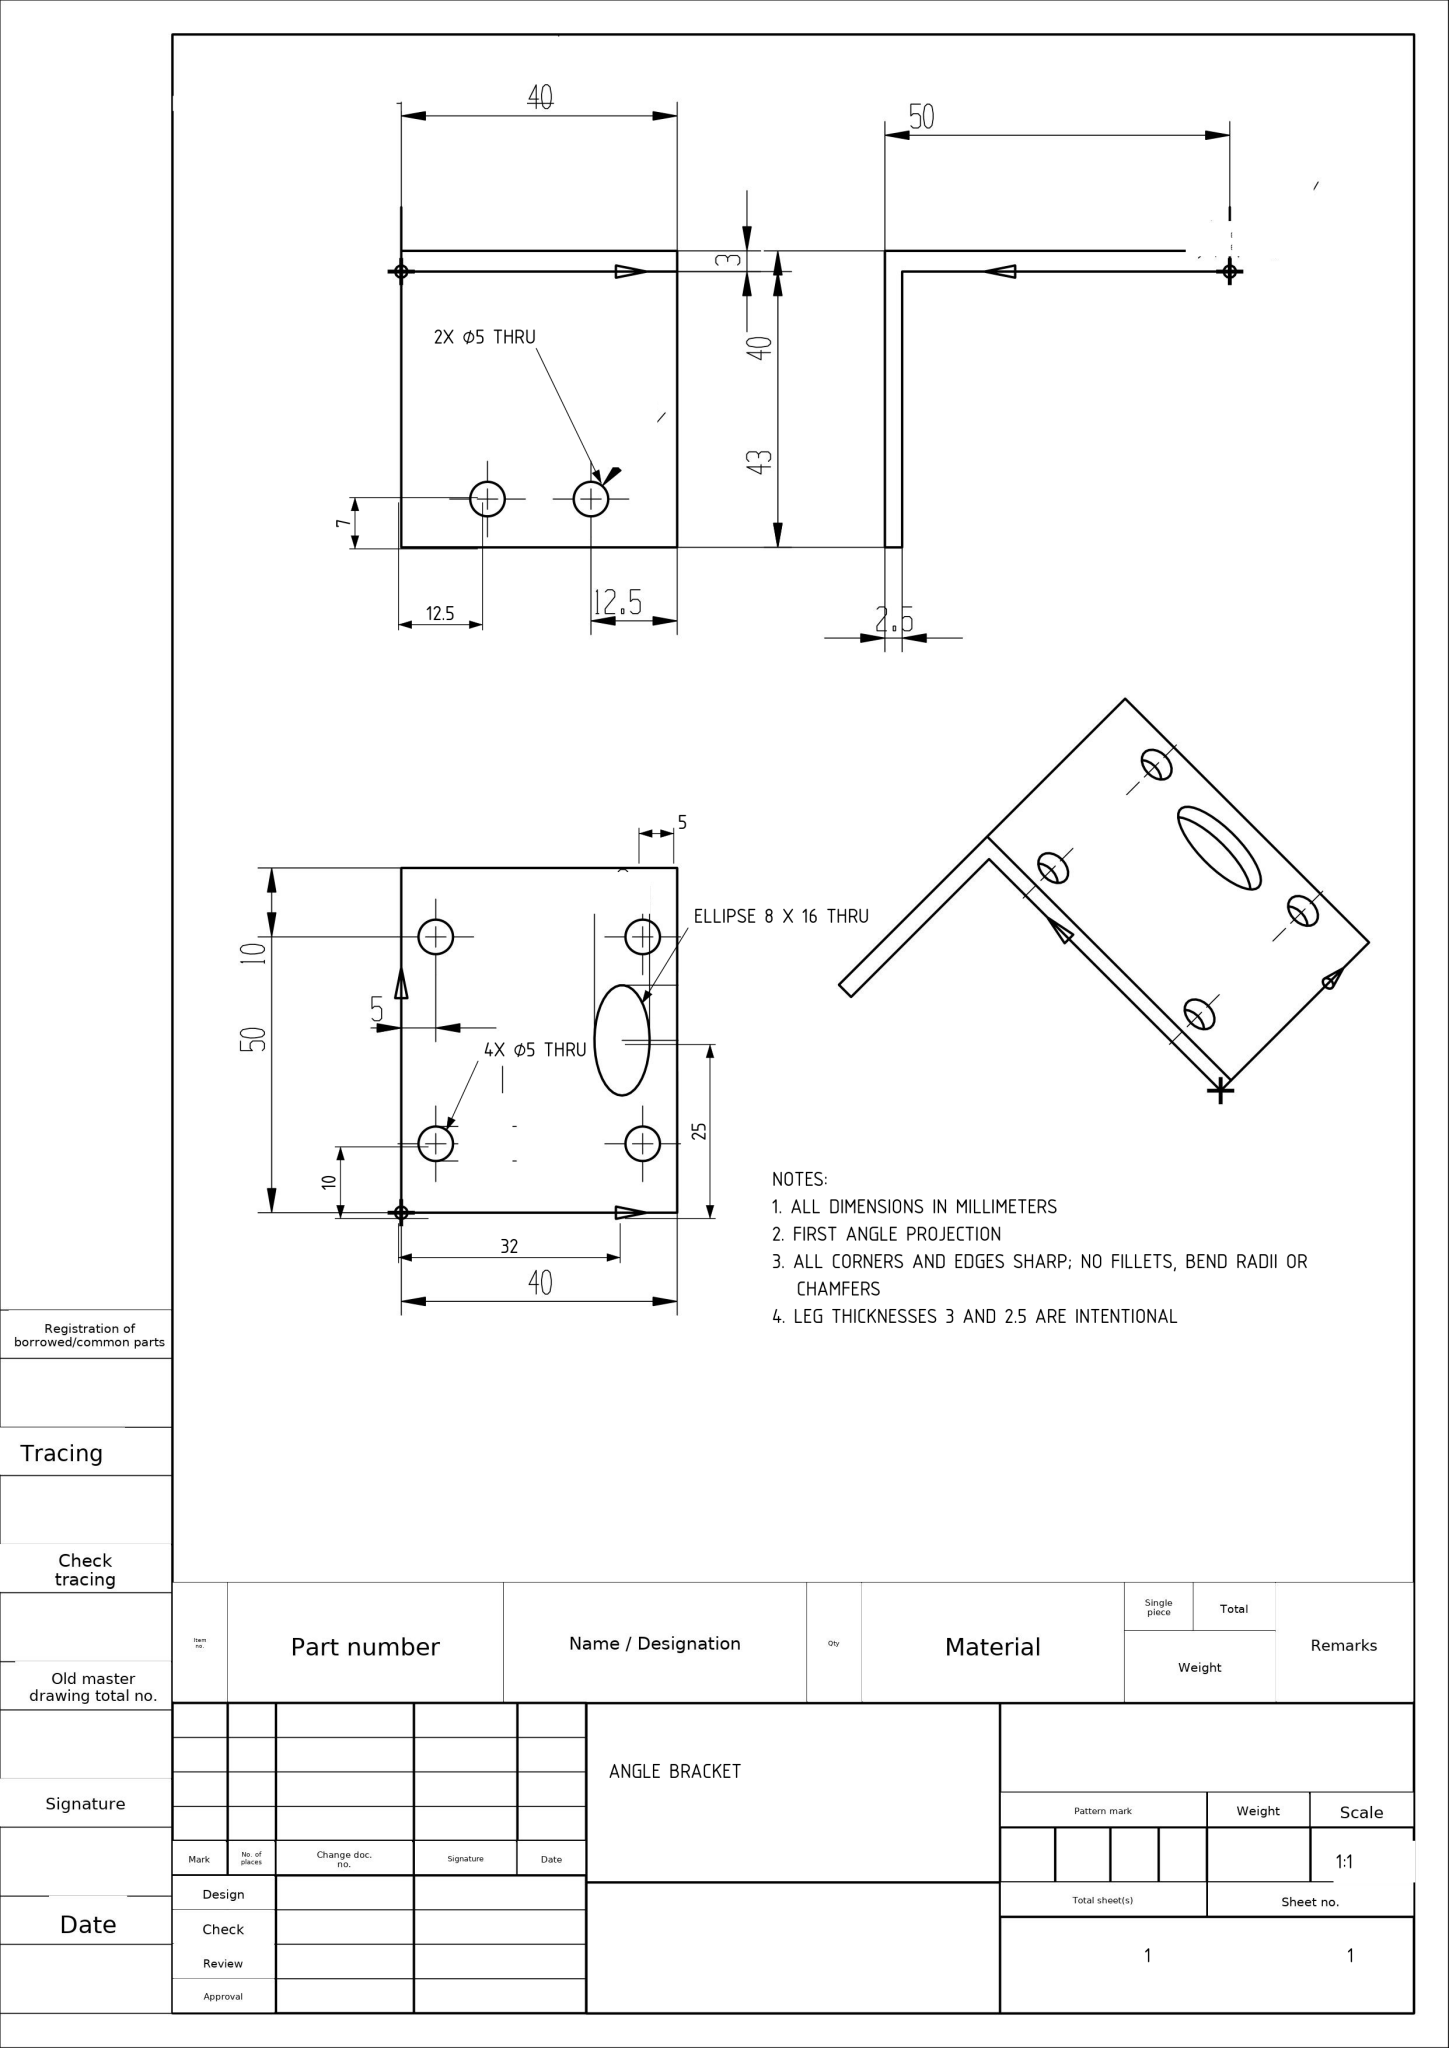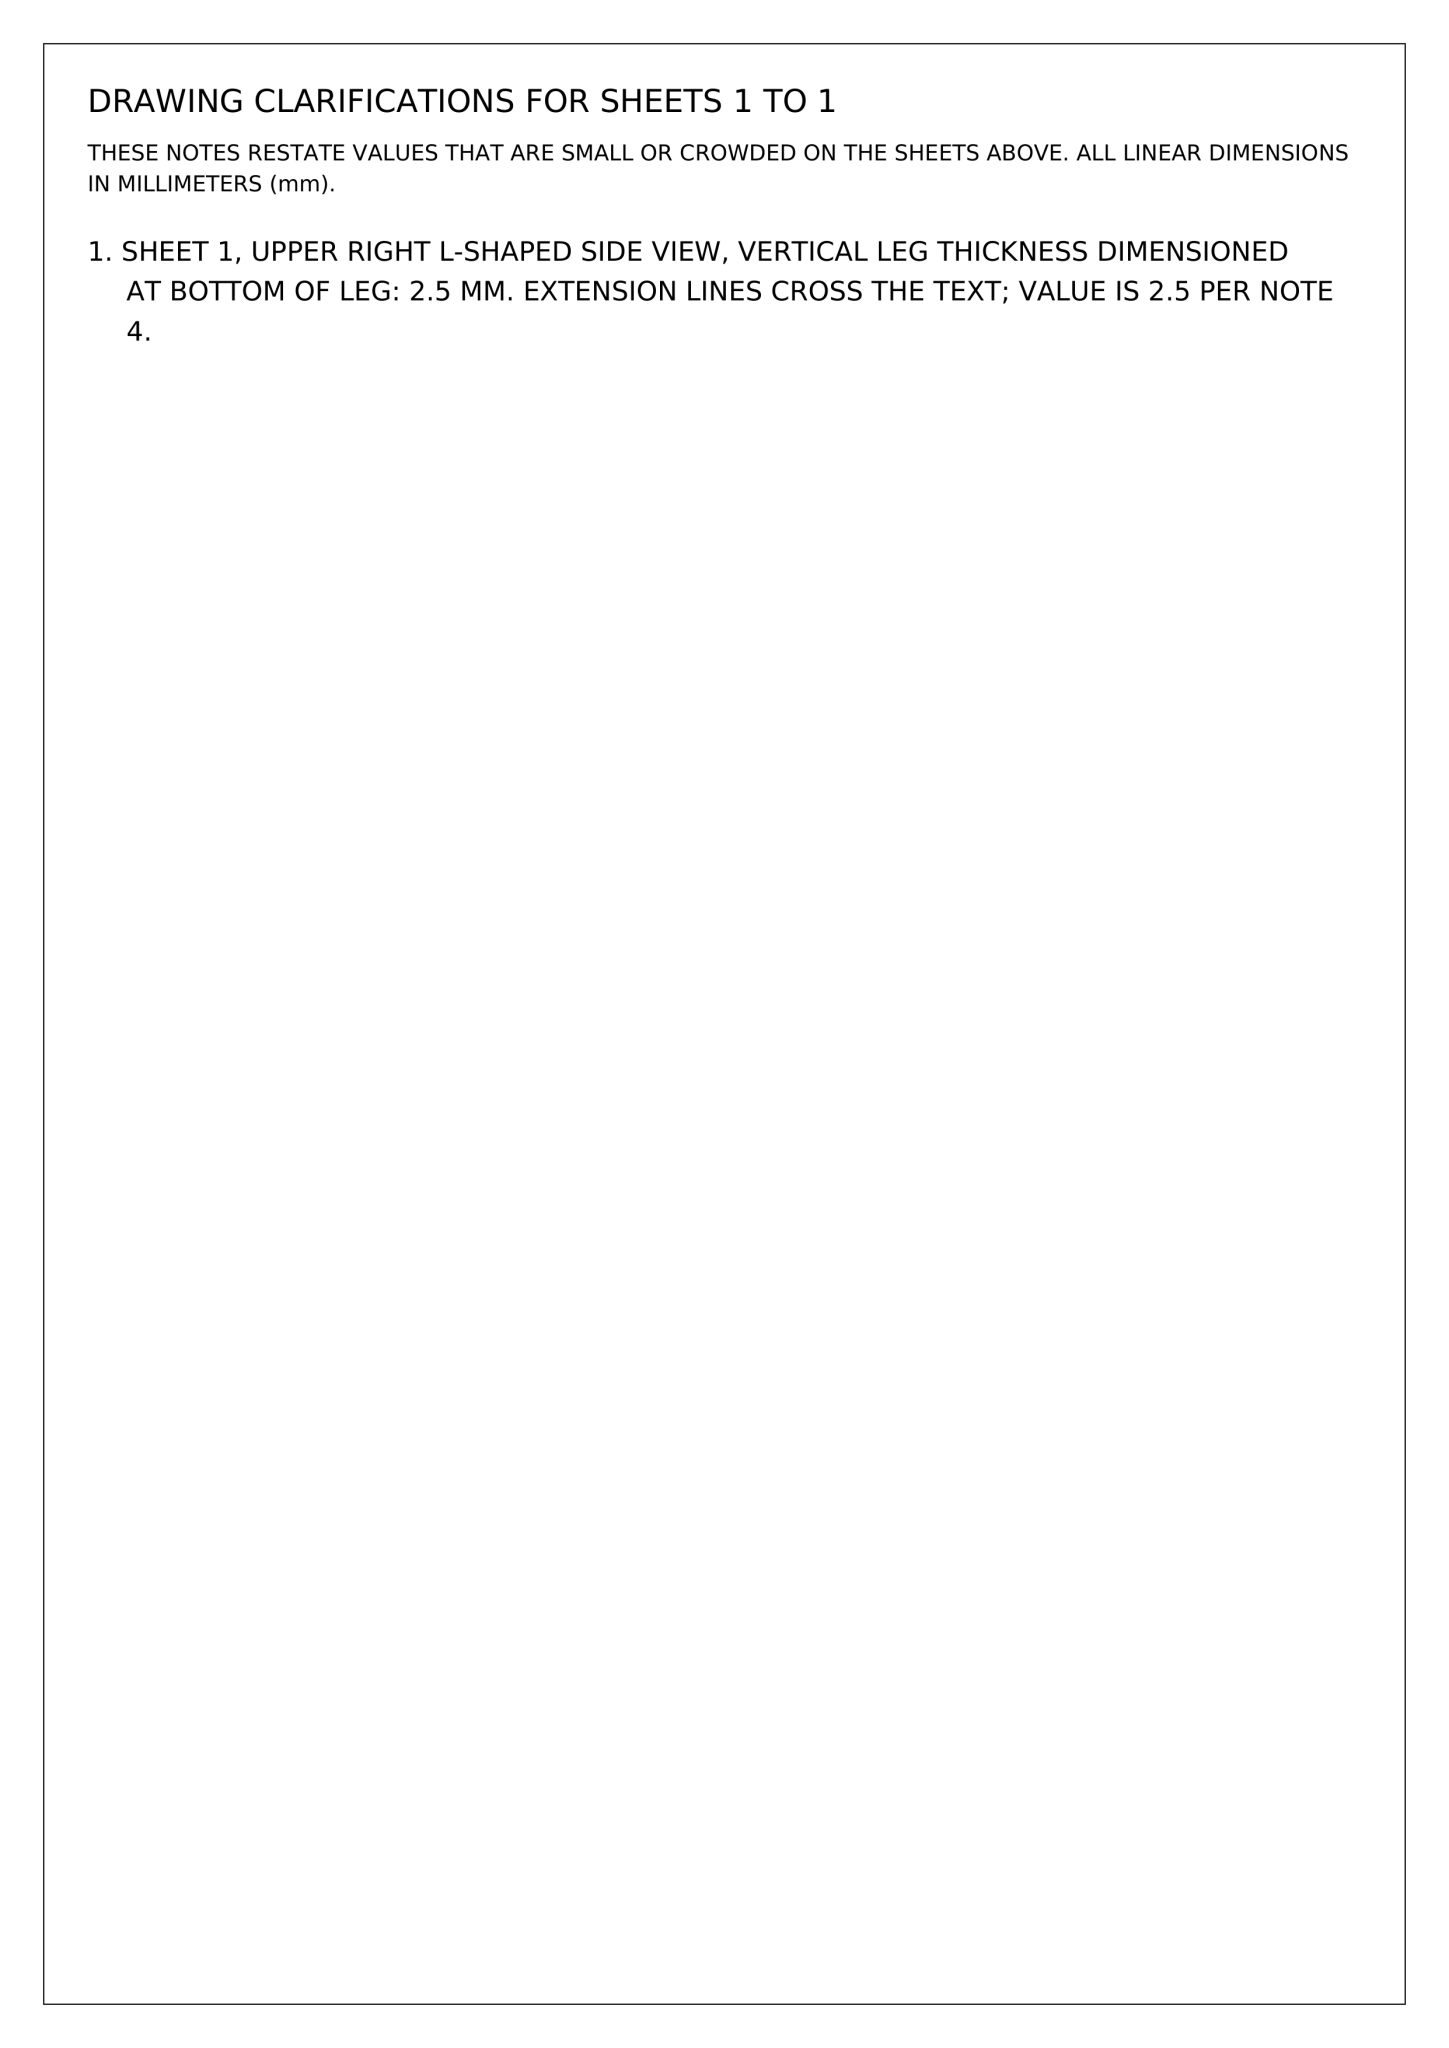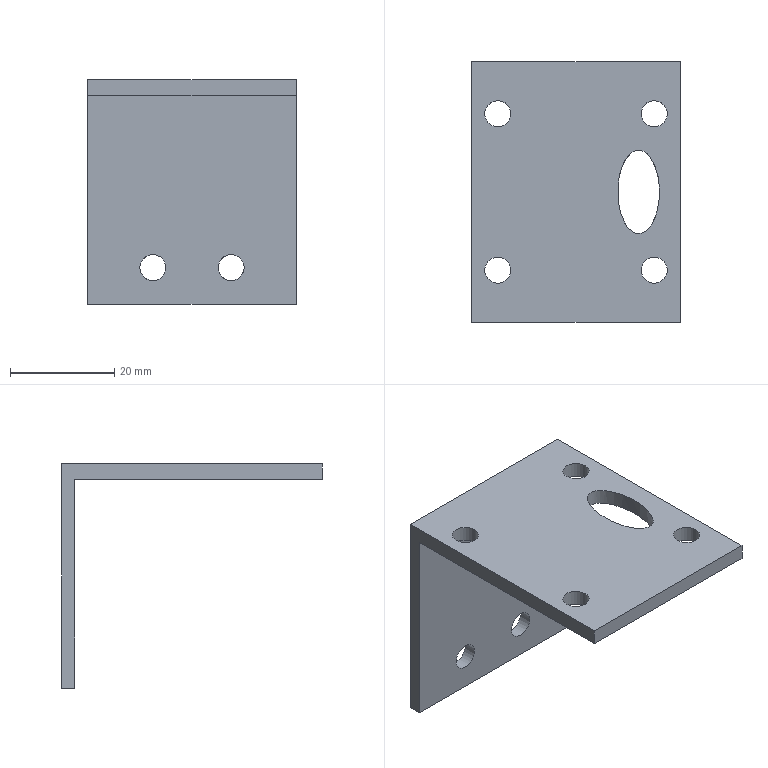Part | NX | mm | 1 solid | 15 faces | box 40 x 50 x 43 mm | volume 9365 mm3 | plane 8 | cylinder 6 | other 1 | commonest cylinder face diameters 5 x6
STEP:
#1=CARTESIAN_POINT('',(0.,0.,0.));
#2=DIRECTION('',(0.,0.,1.));
#3=DIRECTION('',(1.,0.,0.));
#4=AXIS2_PLACEMENT_3D('',#1,#2,#3);
#5=(LENGTH_UNIT()NAMED_UNIT(*)SI_UNIT(.MILLI.,.METRE.));
#6=UNCERTAINTY_MEASURE_WITH_UNIT(LENGTH_MEASURE(0.00002),#5,'','');
#7=(NAMED_UNIT(*)PLANE_ANGLE_UNIT()SI_UNIT($,.RADIAN.));
#8=PLANE_ANGLE_MEASURE_WITH_UNIT(PLANE_ANGLE_MEASURE(0.01745),#7);
#9=DIMENSIONAL_EXPONENTS(0.,0.,0.,0.,0.,0.,0.);
#10=(CONVERSION_BASED_UNIT('',#8)NAMED_UNIT(#9)PLANE_ANGLE_UNIT());
#11=(NAMED_UNIT(*)SI_UNIT($,.STERADIAN.)SOLID_ANGLE_UNIT());
#12=(GEOMETRIC_REPRESENTATION_CONTEXT(3)GLOBAL_UNCERTAINTY_ASSIGNED_CONTEXT((#6))GLOBAL_UNIT_ASSIGNED_CONTEXT((#5,#10,#11))REPRESENTATION_CONTEXT('',''));
#13=SHAPE_REPRESENTATION('',(#4),#12);
#14=CARTESIAN_POINT('',(32.,17.,3.));
#15=VERTEX_POINT('',#14);
#16=CARTESIAN_POINT('',(32.,25.,3.));
#17=DIRECTION('',(0.,0.,1.));
#18=DIRECTION('',(-0.,-1.,0.));
#19=AXIS2_PLACEMENT_3D('',#16,#17,#18);
#20=ELLIPSE('',#19,8.,4.);
#21=EDGE_CURVE('',#15,#15,#20,.T.);
#22=ORIENTED_EDGE('',*,*,#21,.F.);
#23=EDGE_LOOP('',(#22));
#24=FACE_BOUND('',#23,.T.);
#25=CARTESIAN_POINT('',(37.5,40.,3.));
#26=VERTEX_POINT('',#25);
#27=CARTESIAN_POINT('',(35.,40.,3.));
#28=DIRECTION('',(0.,0.,-1.));
#29=DIRECTION('',(1.,0.,0.));
#30=AXIS2_PLACEMENT_3D('',#27,#28,#29);
#31=CIRCLE('',#30,2.5);
#32=EDGE_CURVE('',#26,#26,#31,.T.);
#33=ORIENTED_EDGE('',*,*,#32,.T.);
#34=EDGE_LOOP('',(#33));
#35=FACE_BOUND('',#34,.T.);
#36=CARTESIAN_POINT('',(2.5,10.,3.));
#37=VERTEX_POINT('',#36);
#38=CARTESIAN_POINT('',(5.,10.,3.));
#39=DIRECTION('',(0.,0.,-1.));
#40=DIRECTION('',(-1.,0.,0.));
#41=AXIS2_PLACEMENT_3D('',#38,#39,#40);
#42=CIRCLE('',#41,2.5);
#43=EDGE_CURVE('',#37,#37,#42,.T.);
#44=ORIENTED_EDGE('',*,*,#43,.T.);
#45=EDGE_LOOP('',(#44));
#46=FACE_BOUND('',#45,.T.);
#47=CARTESIAN_POINT('',(40.,0.,3.));
#48=VERTEX_POINT('',#47);
#49=CARTESIAN_POINT('',(0.,0.,3.));
#50=VERTEX_POINT('',#49);
#51=CARTESIAN_POINT('',(20.,0.,3.));
#52=DIRECTION('',(-1.,0.,0.));
#53=VECTOR('',#52,1.);
#54=LINE('',#51,#53);
#55=EDGE_CURVE('',#48,#50,#54,.T.);
#56=ORIENTED_EDGE('',*,*,#55,.F.);
#57=CARTESIAN_POINT('',(40.,50.,3.));
#58=VERTEX_POINT('',#57);
#59=CARTESIAN_POINT('',(40.,25.,3.));
#60=DIRECTION('',(0.,-1.,0.));
#61=VECTOR('',#60,1.);
#62=LINE('',#59,#61);
#63=EDGE_CURVE('',#58,#48,#62,.T.);
#64=ORIENTED_EDGE('',*,*,#63,.F.);
#65=CARTESIAN_POINT('',(0.,50.,3.));
#66=VERTEX_POINT('',#65);
#67=CARTESIAN_POINT('',(20.,50.,3.));
#68=DIRECTION('',(1.,0.,0.));
#69=VECTOR('',#68,1.);
#70=LINE('',#67,#69);
#71=EDGE_CURVE('',#66,#58,#70,.T.);
#72=ORIENTED_EDGE('',*,*,#71,.F.);
#73=CARTESIAN_POINT('',(0.,25.,3.));
#74=DIRECTION('',(0.,1.,0.));
#75=VECTOR('',#74,1.);
#76=LINE('',#73,#75);
#77=EDGE_CURVE('',#50,#66,#76,.T.);
#78=ORIENTED_EDGE('',*,*,#77,.F.);
#79=EDGE_LOOP('',(#56,#64,#72,#78));
#80=FACE_BOUND('',#79,.T.);
#81=CARTESIAN_POINT('',(37.5,10.,3.));
#82=VERTEX_POINT('',#81);
#83=CARTESIAN_POINT('',(35.,10.,3.));
#84=DIRECTION('',(0.,0.,1.));
#85=DIRECTION('',(1.,0.,0.));
#86=AXIS2_PLACEMENT_3D('',#83,#84,#85);
#87=CIRCLE('',#86,2.5);
#88=EDGE_CURVE('',#82,#82,#87,.T.);
#89=ORIENTED_EDGE('',*,*,#88,.F.);
#90=EDGE_LOOP('',(#89));
#91=FACE_BOUND('',#90,.T.);
#92=CARTESIAN_POINT('',(2.5,40.,3.));
#93=VERTEX_POINT('',#92);
#94=CARTESIAN_POINT('',(5.,40.,3.));
#95=DIRECTION('',(0.,0.,1.));
#96=DIRECTION('',(-1.,0.,0.));
#97=AXIS2_PLACEMENT_3D('',#94,#95,#96);
#98=CIRCLE('',#97,2.5);
#99=EDGE_CURVE('',#93,#93,#98,.T.);
#100=ORIENTED_EDGE('',*,*,#99,.F.);
#101=EDGE_LOOP('',(#100));
#102=FACE_BOUND('',#101,.T.);
#103=CARTESIAN_POINT('',(20.,25.,3.));
#104=DIRECTION('',(0.,0.,1.));
#105=DIRECTION('',(1.,0.,0.));
#106=AXIS2_PLACEMENT_3D('',#103,#104,#105);
#107=PLANE('',#106);
#108=ADVANCED_FACE('',(#24,#35,#46,#80,#91,#102),#107,.T.);
#109=CARTESIAN_POINT('',(32.,17.,0.));
#110=VERTEX_POINT('',#109);
#111=CARTESIAN_POINT('',(32.,25.,0.));
#112=DIRECTION('',(0.,0.,-1.));
#113=DIRECTION('',(-0.,-1.,0.));
#114=AXIS2_PLACEMENT_3D('',#111,#112,#113);
#115=ELLIPSE('',#114,8.,4.);
#116=EDGE_CURVE('',#110,#110,#115,.T.);
#117=ORIENTED_EDGE('',*,*,#116,.F.);
#118=EDGE_LOOP('',(#117));
#119=FACE_BOUND('',#118,.T.);
#120=CARTESIAN_POINT('',(40.,47.5,0.));
#121=VERTEX_POINT('',#120);
#122=CARTESIAN_POINT('',(0.,47.5,0.));
#123=VERTEX_POINT('',#122);
#124=CARTESIAN_POINT('',(40.,47.5,0.));
#125=DIRECTION('',(-1.,0.,0.));
#126=VECTOR('',#125,1.);
#127=LINE('',#124,#126);
#128=EDGE_CURVE('',#121,#123,#127,.T.);
#129=ORIENTED_EDGE('',*,*,#128,.F.);
#130=CARTESIAN_POINT('',(40.,0.,0.));
#131=VERTEX_POINT('',#130);
#132=CARTESIAN_POINT('',(40.,25.,0.));
#133=DIRECTION('',(0.,1.,0.));
#134=VECTOR('',#133,1.);
#135=LINE('',#132,#134);
#136=EDGE_CURVE('',#131,#121,#135,.T.);
#137=ORIENTED_EDGE('',*,*,#136,.F.);
#138=CARTESIAN_POINT('',(0.,0.,0.));
#139=VERTEX_POINT('',#138);
#140=CARTESIAN_POINT('',(20.,0.,0.));
#141=DIRECTION('',(1.,0.,0.));
#142=VECTOR('',#141,1.);
#143=LINE('',#140,#142);
#144=EDGE_CURVE('',#139,#131,#143,.T.);
#145=ORIENTED_EDGE('',*,*,#144,.F.);
#146=CARTESIAN_POINT('',(0.,25.,0.));
#147=DIRECTION('',(0.,-1.,0.));
#148=VECTOR('',#147,1.);
#149=LINE('',#146,#148);
#150=EDGE_CURVE('',#123,#139,#149,.T.);
#151=ORIENTED_EDGE('',*,*,#150,.F.);
#152=EDGE_LOOP('',(#129,#137,#145,#151));
#153=FACE_BOUND('',#152,.T.);
#154=CARTESIAN_POINT('',(32.5,40.,0.));
#155=VERTEX_POINT('',#154);
#156=CARTESIAN_POINT('',(35.,40.,0.));
#157=DIRECTION('',(0.,0.,1.));
#158=DIRECTION('',(-1.,0.,0.));
#159=AXIS2_PLACEMENT_3D('',#156,#157,#158);
#160=CIRCLE('',#159,2.5);
#161=EDGE_CURVE('',#155,#155,#160,.T.);
#162=ORIENTED_EDGE('',*,*,#161,.T.);
#163=EDGE_LOOP('',(#162));
#164=FACE_BOUND('',#163,.T.);
#165=CARTESIAN_POINT('',(2.5,10.,0.));
#166=VERTEX_POINT('',#165);
#167=CARTESIAN_POINT('',(5.,10.,0.));
#168=DIRECTION('',(0.,0.,1.));
#169=DIRECTION('',(-1.,0.,0.));
#170=AXIS2_PLACEMENT_3D('',#167,#168,#169);
#171=CIRCLE('',#170,2.5);
#172=EDGE_CURVE('',#166,#166,#171,.T.);
#173=ORIENTED_EDGE('',*,*,#172,.T.);
#174=EDGE_LOOP('',(#173));
#175=FACE_BOUND('',#174,.T.);
#176=CARTESIAN_POINT('',(32.5,10.,0.));
#177=VERTEX_POINT('',#176);
#178=CARTESIAN_POINT('',(35.,10.,0.));
#179=DIRECTION('',(0.,0.,-1.));
#180=DIRECTION('',(-1.,0.,0.));
#181=AXIS2_PLACEMENT_3D('',#178,#179,#180);
#182=CIRCLE('',#181,2.5);
#183=EDGE_CURVE('',#177,#177,#182,.T.);
#184=ORIENTED_EDGE('',*,*,#183,.F.);
#185=EDGE_LOOP('',(#184));
#186=FACE_BOUND('',#185,.T.);
#187=CARTESIAN_POINT('',(2.5,40.,0.));
#188=VERTEX_POINT('',#187);
#189=CARTESIAN_POINT('',(5.,40.,0.));
#190=DIRECTION('',(0.,0.,-1.));
#191=DIRECTION('',(-1.,0.,0.));
#192=AXIS2_PLACEMENT_3D('',#189,#190,#191);
#193=CIRCLE('',#192,2.5);
#194=EDGE_CURVE('',#188,#188,#193,.T.);
#195=ORIENTED_EDGE('',*,*,#194,.F.);
#196=EDGE_LOOP('',(#195));
#197=FACE_BOUND('',#196,.T.);
#198=CARTESIAN_POINT('',(20.,25.,0.));
#199=DIRECTION('',(0.,0.,-1.));
#200=DIRECTION('',(-1.,0.,0.));
#201=AXIS2_PLACEMENT_3D('',#198,#199,#200);
#202=PLANE('',#201);
#203=ADVANCED_FACE('',(#119,#153,#164,#175,#186,#197),#202,.T.);
#204=CARTESIAN_POINT('',(40.,0.,0.));
#205=DIRECTION('',(0.,0.,1.));
#206=VECTOR('',#205,1.);
#207=LINE('',#204,#206);
#208=EDGE_CURVE('',#131,#48,#207,.T.);
#209=ORIENTED_EDGE('',*,*,#208,.T.);
#210=ORIENTED_EDGE('',*,*,#55,.T.);
#211=CARTESIAN_POINT('',(0.,0.,0.));
#212=DIRECTION('',(0.,0.,1.));
#213=VECTOR('',#212,1.);
#214=LINE('',#211,#213);
#215=EDGE_CURVE('',#139,#50,#214,.T.);
#216=ORIENTED_EDGE('',*,*,#215,.F.);
#217=ORIENTED_EDGE('',*,*,#144,.T.);
#218=EDGE_LOOP('',(#209,#210,#216,#217));
#219=FACE_OUTER_BOUND('',#218,.T.);
#220=CARTESIAN_POINT('',(20.,0.,0.));
#221=DIRECTION('',(0.,-1.,0.));
#222=DIRECTION('',(0.,0.,-1.));
#223=AXIS2_PLACEMENT_3D('',#220,#221,#222);
#224=PLANE('',#223);
#225=ADVANCED_FACE('',(#219),#224,.T.);
#226=ORIENTED_EDGE('',*,*,#215,.T.);
#227=ORIENTED_EDGE('',*,*,#77,.T.);
#228=CARTESIAN_POINT('',(0.,50.,-40.));
#229=VERTEX_POINT('',#228);
#230=CARTESIAN_POINT('',(0.,50.,0.));
#231=DIRECTION('',(0.,0.,1.));
#232=VECTOR('',#231,1.);
#233=LINE('',#230,#232);
#234=EDGE_CURVE('',#229,#66,#233,.T.);
#235=ORIENTED_EDGE('',*,*,#234,.F.);
#236=CARTESIAN_POINT('',(0.,47.5,-40.));
#237=VERTEX_POINT('',#236);
#238=CARTESIAN_POINT('',(0.,47.5,-40.));
#239=DIRECTION('',(0.,1.,0.));
#240=VECTOR('',#239,1.);
#241=LINE('',#238,#240);
#242=EDGE_CURVE('',#237,#229,#241,.T.);
#243=ORIENTED_EDGE('',*,*,#242,.F.);
#244=CARTESIAN_POINT('',(0.,47.5,-40.));
#245=DIRECTION('',(0.,0.,1.));
#246=VECTOR('',#245,1.);
#247=LINE('',#244,#246);
#248=EDGE_CURVE('',#237,#123,#247,.T.);
#249=ORIENTED_EDGE('',*,*,#248,.T.);
#250=ORIENTED_EDGE('',*,*,#150,.T.);
#251=EDGE_LOOP('',(#226,#227,#235,#243,#249,#250));
#252=FACE_OUTER_BOUND('',#251,.T.);
#253=CARTESIAN_POINT('',(0.,25.,0.));
#254=DIRECTION('',(-1.,0.,0.));
#255=DIRECTION('',(0.,0.,1.));
#256=AXIS2_PLACEMENT_3D('',#253,#254,#255);
#257=PLANE('',#256);
#258=ADVANCED_FACE('',(#252),#257,.T.);
#259=CARTESIAN_POINT('',(12.5,50.,-30.495));
#260=VERTEX_POINT('',#259);
#261=CARTESIAN_POINT('',(12.5,50.,-32.995));
#262=DIRECTION('',(0.,1.,0.));
#263=DIRECTION('',(0.,0.,1.));
#264=AXIS2_PLACEMENT_3D('',#261,#262,#263);
#265=CIRCLE('',#264,2.5);
#266=EDGE_CURVE('',#260,#260,#265,.T.);
#267=ORIENTED_EDGE('',*,*,#266,.F.);
#268=EDGE_LOOP('',(#267));
#269=FACE_BOUND('',#268,.T.);
#270=CARTESIAN_POINT('',(27.5,50.,-30.495));
#271=VERTEX_POINT('',#270);
#272=CARTESIAN_POINT('',(27.5,50.,-32.995));
#273=DIRECTION('',(0.,1.,0.));
#274=DIRECTION('',(0.,0.,1.));
#275=AXIS2_PLACEMENT_3D('',#272,#273,#274);
#276=CIRCLE('',#275,2.5);
#277=EDGE_CURVE('',#271,#271,#276,.T.);
#278=ORIENTED_EDGE('',*,*,#277,.F.);
#279=EDGE_LOOP('',(#278));
#280=FACE_BOUND('',#279,.T.);
#281=ORIENTED_EDGE('',*,*,#234,.T.);
#282=ORIENTED_EDGE('',*,*,#71,.T.);
#283=CARTESIAN_POINT('',(40.,50.,-40.));
#284=VERTEX_POINT('',#283);
#285=CARTESIAN_POINT('',(40.,50.,0.));
#286=DIRECTION('',(0.,0.,1.));
#287=VECTOR('',#286,1.);
#288=LINE('',#285,#287);
#289=EDGE_CURVE('',#284,#58,#288,.T.);
#290=ORIENTED_EDGE('',*,*,#289,.F.);
#291=CARTESIAN_POINT('',(0.,50.,-40.));
#292=DIRECTION('',(1.,-0.,0.));
#293=VECTOR('',#292,1.);
#294=LINE('',#291,#293);
#295=EDGE_CURVE('',#229,#284,#294,.T.);
#296=ORIENTED_EDGE('',*,*,#295,.F.);
#297=EDGE_LOOP('',(#281,#282,#290,#296));
#298=FACE_BOUND('',#297,.T.);
#299=CARTESIAN_POINT('',(20.,50.,0.));
#300=DIRECTION('',(0.,1.,0.));
#301=DIRECTION('',(0.,0.,1.));
#302=AXIS2_PLACEMENT_3D('',#299,#300,#301);
#303=PLANE('',#302);
#304=ADVANCED_FACE('',(#269,#280,#298),#303,.T.);
#305=ORIENTED_EDGE('',*,*,#136,.T.);
#306=CARTESIAN_POINT('',(40.,47.5,-40.));
#307=VERTEX_POINT('',#306);
#308=CARTESIAN_POINT('',(40.,47.5,-40.));
#309=DIRECTION('',(0.,0.,1.));
#310=VECTOR('',#309,1.);
#311=LINE('',#308,#310);
#312=EDGE_CURVE('',#307,#121,#311,.T.);
#313=ORIENTED_EDGE('',*,*,#312,.F.);
#314=CARTESIAN_POINT('',(40.,50.,-40.));
#315=DIRECTION('',(0.,-1.,0.));
#316=VECTOR('',#315,1.);
#317=LINE('',#314,#316);
#318=EDGE_CURVE('',#284,#307,#317,.T.);
#319=ORIENTED_EDGE('',*,*,#318,.F.);
#320=ORIENTED_EDGE('',*,*,#289,.T.);
#321=ORIENTED_EDGE('',*,*,#63,.T.);
#322=ORIENTED_EDGE('',*,*,#208,.F.);
#323=EDGE_LOOP('',(#305,#313,#319,#320,#321,#322));
#324=FACE_OUTER_BOUND('',#323,.T.);
#325=CARTESIAN_POINT('',(40.,25.,0.));
#326=DIRECTION('',(1.,0.,0.));
#327=DIRECTION('',(0.,0.,-1.));
#328=AXIS2_PLACEMENT_3D('',#325,#326,#327);
#329=PLANE('',#328);
#330=ADVANCED_FACE('',(#324),#329,.T.);
#331=ORIENTED_EDGE('',*,*,#172,.F.);
#332=EDGE_LOOP('',(#331));
#333=FACE_BOUND('',#332,.T.);
#334=ORIENTED_EDGE('',*,*,#43,.F.);
#335=EDGE_LOOP('',(#334));
#336=FACE_BOUND('',#335,.T.);
#337=CARTESIAN_POINT('',(5.,10.,-32.));
#338=DIRECTION('',(0.,0.,1.));
#339=DIRECTION('',(1.,0.,0.));
#340=AXIS2_PLACEMENT_3D('',#337,#338,#339);
#341=CYLINDRICAL_SURFACE('',#340,2.5);
#342=ADVANCED_FACE('',(#333,#336),#341,.F.);
#343=ORIENTED_EDGE('',*,*,#161,.F.);
#344=EDGE_LOOP('',(#343));
#345=FACE_BOUND('',#344,.T.);
#346=ORIENTED_EDGE('',*,*,#32,.F.);
#347=EDGE_LOOP('',(#346));
#348=FACE_BOUND('',#347,.T.);
#349=CARTESIAN_POINT('',(35.,40.,-32.));
#350=DIRECTION('',(0.,0.,1.));
#351=DIRECTION('',(1.,0.,0.));
#352=AXIS2_PLACEMENT_3D('',#349,#350,#351);
#353=CYLINDRICAL_SURFACE('',#352,2.5);
#354=ADVANCED_FACE('',(#345,#348),#353,.F.);
#355=ORIENTED_EDGE('',*,*,#183,.T.);
#356=EDGE_LOOP('',(#355));
#357=FACE_BOUND('',#356,.T.);
#358=ORIENTED_EDGE('',*,*,#88,.T.);
#359=EDGE_LOOP('',(#358));
#360=FACE_BOUND('',#359,.T.);
#361=CARTESIAN_POINT('',(35.,10.,-32.));
#362=DIRECTION('',(0.,0.,1.));
#363=DIRECTION('',(1.,0.,0.));
#364=AXIS2_PLACEMENT_3D('',#361,#362,#363);
#365=CYLINDRICAL_SURFACE('',#364,2.5);
#366=ADVANCED_FACE('',(#357,#360),#365,.F.);
#367=ORIENTED_EDGE('',*,*,#194,.T.);
#368=EDGE_LOOP('',(#367));
#369=FACE_BOUND('',#368,.T.);
#370=ORIENTED_EDGE('',*,*,#99,.T.);
#371=EDGE_LOOP('',(#370));
#372=FACE_BOUND('',#371,.T.);
#373=CARTESIAN_POINT('',(5.,40.,-32.));
#374=DIRECTION('',(0.,0.,1.));
#375=DIRECTION('',(1.,0.,0.));
#376=AXIS2_PLACEMENT_3D('',#373,#374,#375);
#377=CYLINDRICAL_SURFACE('',#376,2.5);
#378=ADVANCED_FACE('',(#369,#372),#377,.F.);
#379=CARTESIAN_POINT('',(15.,47.5,-32.995));
#380=VERTEX_POINT('',#379);
#381=CARTESIAN_POINT('',(12.5,47.5,-32.995));
#382=DIRECTION('',(0.,-1.,0.));
#383=DIRECTION('',(1.,0.,0.));
#384=AXIS2_PLACEMENT_3D('',#381,#382,#383);
#385=CIRCLE('',#384,2.5);
#386=EDGE_CURVE('',#380,#380,#385,.T.);
#387=ORIENTED_EDGE('',*,*,#386,.F.);
#388=EDGE_LOOP('',(#387));
#389=FACE_BOUND('',#388,.T.);
#390=CARTESIAN_POINT('',(30.,47.5,-32.995));
#391=VERTEX_POINT('',#390);
#392=CARTESIAN_POINT('',(27.5,47.5,-32.995));
#393=DIRECTION('',(0.,-1.,0.));
#394=DIRECTION('',(1.,0.,0.));
#395=AXIS2_PLACEMENT_3D('',#392,#393,#394);
#396=CIRCLE('',#395,2.5);
#397=EDGE_CURVE('',#391,#391,#396,.T.);
#398=ORIENTED_EDGE('',*,*,#397,.F.);
#399=EDGE_LOOP('',(#398));
#400=FACE_BOUND('',#399,.T.);
#401=ORIENTED_EDGE('',*,*,#128,.T.);
#402=ORIENTED_EDGE('',*,*,#248,.F.);
#403=CARTESIAN_POINT('',(40.,47.5,-40.));
#404=DIRECTION('',(-1.,0.,0.));
#405=VECTOR('',#404,1.);
#406=LINE('',#403,#405);
#407=EDGE_CURVE('',#307,#237,#406,.T.);
#408=ORIENTED_EDGE('',*,*,#407,.F.);
#409=ORIENTED_EDGE('',*,*,#312,.T.);
#410=EDGE_LOOP('',(#401,#402,#408,#409));
#411=FACE_BOUND('',#410,.T.);
#412=CARTESIAN_POINT('',(40.,47.5,-40.));
#413=DIRECTION('',(0.,1.,0.));
#414=DIRECTION('',(-1.,0.,0.));
#415=AXIS2_PLACEMENT_3D('',#412,#413,#414);
#416=PLANE('',#415);
#417=ADVANCED_FACE('',(#389,#400,#411),#416,.F.);
#418=ORIENTED_EDGE('',*,*,#242,.T.);
#419=ORIENTED_EDGE('',*,*,#295,.T.);
#420=ORIENTED_EDGE('',*,*,#318,.T.);
#421=ORIENTED_EDGE('',*,*,#407,.T.);
#422=EDGE_LOOP('',(#418,#419,#420,#421));
#423=FACE_OUTER_BOUND('',#422,.T.);
#424=CARTESIAN_POINT('',(0.,0.,-40.));
#425=DIRECTION('',(0.,0.,-1.));
#426=DIRECTION('',(-1.,0.,0.));
#427=AXIS2_PLACEMENT_3D('',#424,#425,#426);
#428=PLANE('',#427);
#429=ADVANCED_FACE('',(#423),#428,.T.);
#430=ORIENTED_EDGE('',*,*,#116,.T.);
#431=EDGE_LOOP('',(#430));
#432=FACE_BOUND('',#431,.T.);
#433=ORIENTED_EDGE('',*,*,#21,.T.);
#434=EDGE_LOOP('',(#433));
#435=FACE_BOUND('',#434,.T.);
#436=CARTESIAN_POINT('',(32.,25.,-57.));
#437=DIRECTION('',(0.,0.,1.));
#438=DIRECTION('',(-0.,-1.,0.));
#439=AXIS2_PLACEMENT_3D('',#436,#437,#438);
#440=ELLIPSE('',#439,8.,4.);
#441=DIRECTION('',(0.,0.,1.));
#442=VECTOR('',#441,1.);
#443=SURFACE_OF_LINEAR_EXTRUSION('',#440,#442);
#444=ADVANCED_FACE('',(#432,#435),#443,.F.);
#445=ORIENTED_EDGE('',*,*,#277,.T.);
#446=EDGE_LOOP('',(#445));
#447=FACE_BOUND('',#446,.T.);
#448=ORIENTED_EDGE('',*,*,#397,.T.);
#449=EDGE_LOOP('',(#448));
#450=FACE_BOUND('',#449,.T.);
#451=CARTESIAN_POINT('',(27.5,61.5,-32.995));
#452=DIRECTION('',(0.,-1.,0.));
#453=DIRECTION('',(0.,0.,-1.));
#454=AXIS2_PLACEMENT_3D('',#451,#452,#453);
#455=CYLINDRICAL_SURFACE('',#454,2.5);
#456=ADVANCED_FACE('',(#447,#450),#455,.F.);
#457=ORIENTED_EDGE('',*,*,#266,.T.);
#458=EDGE_LOOP('',(#457));
#459=FACE_BOUND('',#458,.T.);
#460=ORIENTED_EDGE('',*,*,#386,.T.);
#461=EDGE_LOOP('',(#460));
#462=FACE_BOUND('',#461,.T.);
#463=CARTESIAN_POINT('',(12.5,61.5,-32.995));
#464=DIRECTION('',(0.,-1.,0.));
#465=DIRECTION('',(0.,0.,-1.));
#466=AXIS2_PLACEMENT_3D('',#463,#464,#465);
#467=CYLINDRICAL_SURFACE('',#466,2.5);
#468=ADVANCED_FACE('',(#459,#462),#467,.F.);
#469=CLOSED_SHELL('',(#108,#203,#225,#258,#304,#330,#342,#354,#366,#378,#417,#429,#444,#456,#468));
#470=MANIFOLD_SOLID_BREP('',#469);
#471=ADVANCED_BREP_SHAPE_REPRESENTATION('',(#470),#12);
#472=SHAPE_REPRESENTATION_RELATIONSHIP('','',#13,#471);
#473=PRESENTATION_LAYER_ASSIGNMENT('','',(#470));
#474=COLOUR_RGB('',0.6941,0.6941,0.6941);
#475=FILL_AREA_STYLE_COLOUR('',#474);
#476=FILL_AREA_STYLE('',(#475));
#477=SURFACE_STYLE_FILL_AREA(#476);
#478=SURFACE_SIDE_STYLE('',(#477));
#479=SURFACE_STYLE_USAGE(.BOTH.,#478);
#480=PRESENTATION_STYLE_ASSIGNMENT((#479));
#481=STYLED_ITEM('',(#480),#470);
#482=MECHANICAL_DESIGN_GEOMETRIC_PRESENTATION_REPRESENTATION('',(#481),#12);